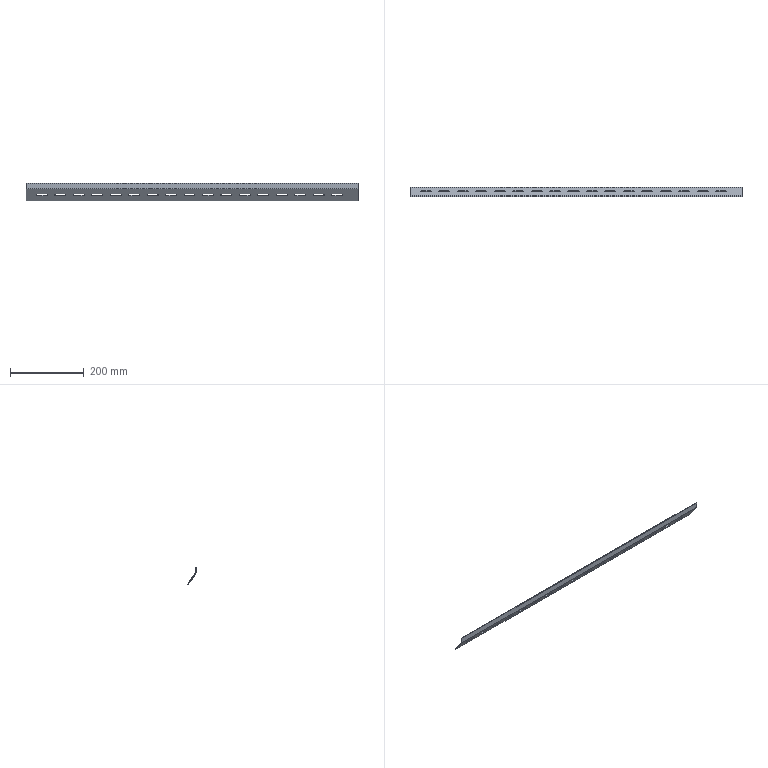Component | SolidWorks | TerminalPlate-1 | 1 solid | 76 faces | volume 91082 mm3 | plane 42 | cylinder 34 | commonest cylinder face diameters 7 x34